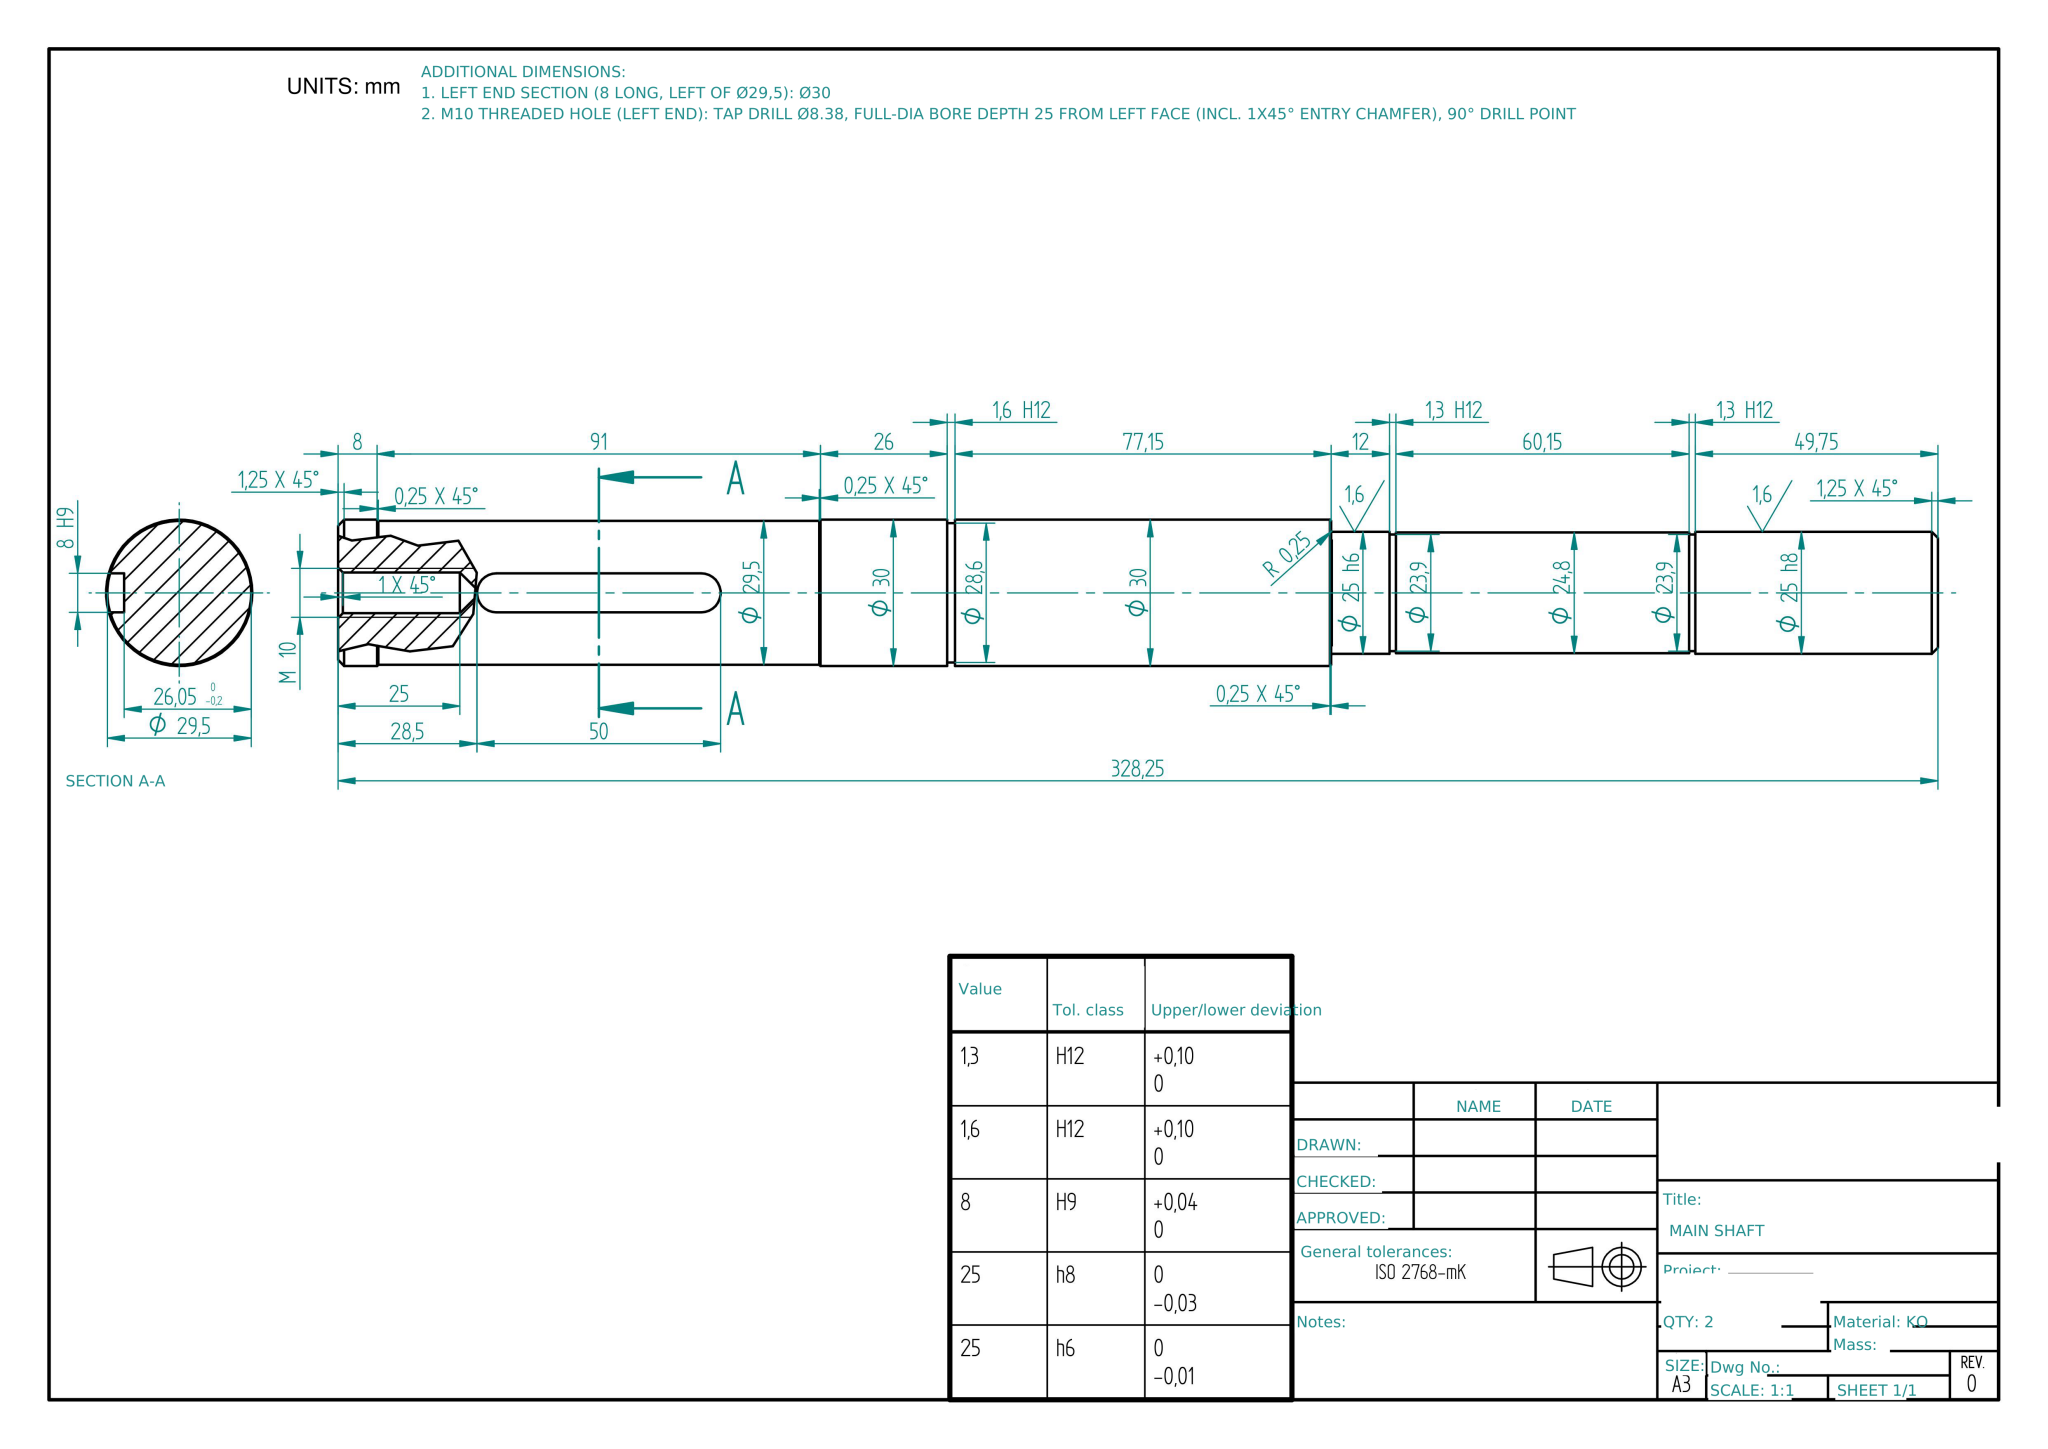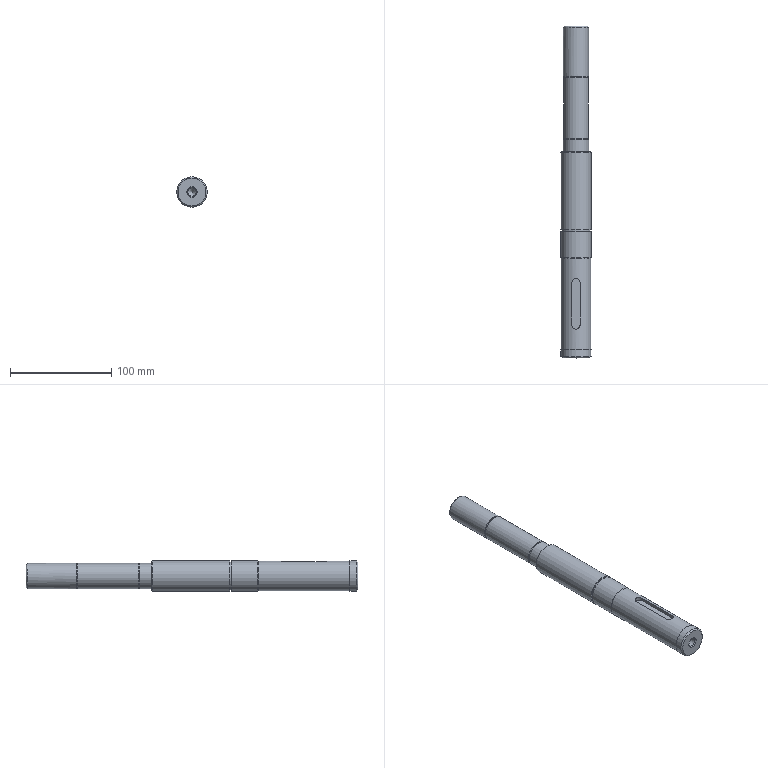Part | NX | mm | 1 solid | 33 faces | box 30 x 328.25 x 30 mm | volume 199467 mm3 | cylinder 13 | plane 12 | cone 7 | torus 1 | commonest cylinder face diameters 30 x3 8 x2 25 x2 23.9 x2 8.376 x1 29.5 x1 24.8 x1 28.6 x1
STEP:
#1=VALUE_REPRESENTATION_ITEM('',COUNT_MEASURE(0.));
#2=(LENGTH_UNIT()NAMED_UNIT(*)SI_UNIT(.MILLI.,.METRE.));
#3=UNCERTAINTY_MEASURE_WITH_UNIT(LENGTH_MEASURE(0.005),#2,'','');
#4=(NAMED_UNIT(*)PLANE_ANGLE_UNIT()SI_UNIT($,.RADIAN.));
#5=(NAMED_UNIT(*)SI_UNIT($,.STERADIAN.)SOLID_ANGLE_UNIT());
#6=(GEOMETRIC_REPRESENTATION_CONTEXT(3)GLOBAL_UNCERTAINTY_ASSIGNED_CONTEXT((#3))GLOBAL_UNIT_ASSIGNED_CONTEXT((#2,#4,#5))REPRESENTATION_CONTEXT('',''));
#7=REPRESENTATION('',(#1),#6);
#8=VALUE_REPRESENTATION_ITEM('',COUNT_MEASURE(0.));
#9=REPRESENTATION('',(#8),#6);
#10=CARTESIAN_POINT('',(0.,0.,0.));
#11=DIRECTION('',(0.,0.,1.));
#12=DIRECTION('',(1.,0.,0.));
#13=AXIS2_PLACEMENT_3D('',#10,#11,#12);
#14=SHAPE_REPRESENTATION('',(#13),#6);
#15=CARTESIAN_POINT('',(0.,-28.5,4.188));
#16=VERTEX_POINT('',#15);
#17=CARTESIAN_POINT('',(0.,-28.5,-0.));
#18=DIRECTION('',(0.,1.,0.));
#19=DIRECTION('',(0.,0.,1.));
#20=AXIS2_PLACEMENT_3D('',#17,#18,#19);
#21=CIRCLE('',#20,4.188);
#22=EDGE_CURVE('',#16,#16,#21,.T.);
#23=ORIENTED_EDGE('',*,*,#22,.F.);
#24=EDGE_LOOP('',(#23));
#25=FACE_BOUND('',#24,.T.);
#26=CARTESIAN_POINT('',(0.,-24.312,-0.));
#27=VERTEX_POINT('',#26);
#28=VERTEX_LOOP('',#27);
#29=FACE_BOUND('',#28,.T.);
#30=CARTESIAN_POINT('',(0.,-28.5,-0.));
#31=DIRECTION('',(0.,-1.,0.));
#32=DIRECTION('',(0.,0.,1.));
#33=AXIS2_PLACEMENT_3D('',#30,#31,#32);
#34=CONICAL_SURFACE('',#33,4.188,0.7854);
#35=ADVANCED_FACE('',(#25,#29),#34,.F.);
#36=CARTESIAN_POINT('',(0.,-53.5,5.188));
#37=VERTEX_POINT('',#36);
#38=CARTESIAN_POINT('',(0.,-53.5,-0.));
#39=DIRECTION('',(0.,1.,0.));
#40=DIRECTION('',(0.,0.,1.));
#41=AXIS2_PLACEMENT_3D('',#38,#39,#40);
#42=CIRCLE('',#41,5.188);
#43=EDGE_CURVE('',#37,#37,#42,.T.);
#44=ORIENTED_EDGE('',*,*,#43,.F.);
#45=EDGE_LOOP('',(#44));
#46=FACE_BOUND('',#45,.T.);
#47=CARTESIAN_POINT('',(0.,-52.5,4.188));
#48=VERTEX_POINT('',#47);
#49=CARTESIAN_POINT('',(0.,-52.5,-0.));
#50=DIRECTION('',(0.,-1.,0.));
#51=DIRECTION('',(0.,0.,1.));
#52=AXIS2_PLACEMENT_3D('',#49,#50,#51);
#53=CIRCLE('',#52,4.188);
#54=EDGE_CURVE('',#48,#48,#53,.T.);
#55=ORIENTED_EDGE('',*,*,#54,.F.);
#56=EDGE_LOOP('',(#55));
#57=FACE_BOUND('',#56,.T.);
#58=CARTESIAN_POINT('',(0.,-53.5,-0.));
#59=DIRECTION('',(0.,-1.,0.));
#60=DIRECTION('',(0.,0.,-1.));
#61=AXIS2_PLACEMENT_3D('',#58,#59,#60);
#62=CONICAL_SURFACE('',#61,5.188,0.7854);
#63=ADVANCED_FACE('',(#46,#57),#62,.F.);
#64=ORIENTED_EDGE('',*,*,#54,.T.);
#65=EDGE_LOOP('',(#64));
#66=FACE_BOUND('',#65,.T.);
#67=ORIENTED_EDGE('',*,*,#22,.T.);
#68=EDGE_LOOP('',(#67));
#69=FACE_BOUND('',#68,.T.);
#70=CARTESIAN_POINT('',(0.,-53.5,-0.));
#71=DIRECTION('',(0.,-1.,0.));
#72=DIRECTION('',(0.,0.,-1.));
#73=AXIS2_PLACEMENT_3D('',#70,#71,#72);
#74=CYLINDRICAL_SURFACE('',#73,4.188);
#75=ADVANCED_FACE('',(#66,#69),#74,.F.);
#76=CARTESIAN_POINT('',(-0.,-45.25,-14.75));
#77=VERTEX_POINT('',#76);
#78=CARTESIAN_POINT('',(-0.,-45.25,0.));
#79=DIRECTION('',(-0.,-1.,-0.));
#80=DIRECTION('',(0.,0.,-1.));
#81=AXIS2_PLACEMENT_3D('',#78,#79,#80);
#82=CIRCLE('',#81,14.75);
#83=EDGE_CURVE('',#77,#77,#82,.T.);
#84=ORIENTED_EDGE('',*,*,#83,.F.);
#85=EDGE_LOOP('',(#84));
#86=FACE_BOUND('',#85,.T.);
#87=CARTESIAN_POINT('',(0.,45.25,-14.75));
#88=VERTEX_POINT('',#87);
#89=CARTESIAN_POINT('',(0.,45.25,0.));
#90=DIRECTION('',(-0.,-1.,-0.));
#91=DIRECTION('',(0.,0.,-1.));
#92=AXIS2_PLACEMENT_3D('',#89,#90,#91);
#93=CIRCLE('',#92,14.75);
#94=EDGE_CURVE('',#88,#88,#93,.T.);
#95=ORIENTED_EDGE('',*,*,#94,.T.);
#96=EDGE_LOOP('',(#95));
#97=FACE_BOUND('',#96,.T.);
#98=CARTESIAN_POINT('',(-4.,21.,14.197));
#99=VERTEX_POINT('',#98);
#100=CARTESIAN_POINT('',(-4.,-21.,14.197));
#101=VERTEX_POINT('',#100);
#102=CARTESIAN_POINT('',(-4.,-60.,14.197));
#103=DIRECTION('',(-0.,-1.,-0.));
#104=VECTOR('',#103,1000.);
#105=LINE('',#102,#104);
#106=EDGE_CURVE('',#99,#101,#105,.T.);
#107=ORIENTED_EDGE('',*,*,#106,.F.);
#108=CARTESIAN_POINT('',(4.,21.,14.197));
#109=VERTEX_POINT('',#108);
#110=CARTESIAN_POINT('',(-4.,21.,14.197));
#111=CARTESIAN_POINT('',(-4.,22.062,14.197));
#112=CARTESIAN_POINT('',(-3.133,24.126,14.479));
#113=CARTESIAN_POINT('',(-0.005917,25.437,14.885));
#114=CARTESIAN_POINT('',(3.134,24.128,14.479));
#115=CARTESIAN_POINT('',(4.,22.062,14.197));
#116=CARTESIAN_POINT('',(4.,21.,14.197));
#117=B_SPLINE_CURVE_WITH_KNOTS('',3,(#110,#111,#112,#113,#114,#115,#116),.UNSPECIFIED.,.F.,.F.,(4,1,1,1,4),(0.,0.00314,0.00628,0.009421,0.01256),.UNSPECIFIED.);
#118=EDGE_CURVE('',#99,#109,#117,.T.);
#119=ORIENTED_EDGE('',*,*,#118,.T.);
#120=CARTESIAN_POINT('',(4.,-21.,14.197));
#121=VERTEX_POINT('',#120);
#122=CARTESIAN_POINT('',(4.,-60.,14.197));
#123=DIRECTION('',(0.,1.,0.));
#124=VECTOR('',#123,1000.);
#125=LINE('',#122,#124);
#126=EDGE_CURVE('',#121,#109,#125,.T.);
#127=ORIENTED_EDGE('',*,*,#126,.F.);
#128=CARTESIAN_POINT('',(4.,-21.,14.197));
#129=CARTESIAN_POINT('',(4.,-22.062,14.197));
#130=CARTESIAN_POINT('',(3.133,-24.126,14.479));
#131=CARTESIAN_POINT('',(0.005917,-25.437,14.885));
#132=CARTESIAN_POINT('',(-3.134,-24.128,14.479));
#133=CARTESIAN_POINT('',(-4.,-22.062,14.197));
#134=CARTESIAN_POINT('',(-4.,-21.,14.197));
#135=B_SPLINE_CURVE_WITH_KNOTS('',3,(#128,#129,#130,#131,#132,#133,#134),.UNSPECIFIED.,.F.,.F.,(4,1,1,1,4),(0.,0.00314,0.00628,0.009421,0.01256),.UNSPECIFIED.);
#136=EDGE_CURVE('',#121,#101,#135,.T.);
#137=ORIENTED_EDGE('',*,*,#136,.T.);
#138=EDGE_LOOP('',(#107,#119,#127,#137));
#139=FACE_BOUND('',#138,.T.);
#140=CARTESIAN_POINT('',(-0.,-60.,0.));
#141=DIRECTION('',(0.,1.,0.));
#142=DIRECTION('',(0.,0.,-1.));
#143=AXIS2_PLACEMENT_3D('',#140,#141,#142);
#144=CYLINDRICAL_SURFACE('',#143,14.75);
#145=ADVANCED_FACE('',(#86,#97,#139),#144,.T.);
#146=ORIENTED_EDGE('',*,*,#136,.F.);
#147=CARTESIAN_POINT('',(4.,-21.,11.3));
#148=VERTEX_POINT('',#147);
#149=CARTESIAN_POINT('',(4.,-21.,14.197));
#150=DIRECTION('',(0.,0.,1.));
#151=VECTOR('',#150,1000.);
#152=LINE('',#149,#151);
#153=EDGE_CURVE('',#148,#121,#152,.T.);
#154=ORIENTED_EDGE('',*,*,#153,.F.);
#155=CARTESIAN_POINT('',(-4.,-21.,11.3));
#156=VERTEX_POINT('',#155);
#157=CARTESIAN_POINT('',(0.,-21.,11.3));
#158=DIRECTION('',(0.,0.,1.));
#159=DIRECTION('',(1.,0.,0.));
#160=AXIS2_PLACEMENT_3D('',#157,#158,#159);
#161=CIRCLE('',#160,4.);
#162=EDGE_CURVE('',#156,#148,#161,.T.);
#163=ORIENTED_EDGE('',*,*,#162,.F.);
#164=CARTESIAN_POINT('',(-4.,-21.,11.3));
#165=DIRECTION('',(0.,0.,-1.));
#166=VECTOR('',#165,1000.);
#167=LINE('',#164,#166);
#168=EDGE_CURVE('',#101,#156,#167,.T.);
#169=ORIENTED_EDGE('',*,*,#168,.F.);
#170=EDGE_LOOP('',(#146,#154,#163,#169));
#171=FACE_BOUND('',#170,.T.);
#172=CARTESIAN_POINT('',(0.,-21.,270.792));
#173=DIRECTION('',(0.,0.,-1.));
#174=DIRECTION('',(1.,0.,0.));
#175=AXIS2_PLACEMENT_3D('',#172,#173,#174);
#176=CYLINDRICAL_SURFACE('',#175,4.);
#177=ADVANCED_FACE('',(#171),#176,.F.);
#178=CARTESIAN_POINT('',(0.,273.5,-12.5));
#179=VERTEX_POINT('',#178);
#180=CARTESIAN_POINT('',(0.,273.5,0.));
#181=DIRECTION('',(0.,-1.,0.));
#182=DIRECTION('',(0.,0.,-1.));
#183=AXIS2_PLACEMENT_3D('',#180,#181,#182);
#184=CIRCLE('',#183,12.5);
#185=EDGE_CURVE('',#179,#179,#184,.T.);
#186=ORIENTED_EDGE('',*,*,#185,.F.);
#187=EDGE_LOOP('',(#186));
#188=FACE_BOUND('',#187,.T.);
#189=CARTESIAN_POINT('',(0.,274.75,-11.25));
#190=VERTEX_POINT('',#189);
#191=CARTESIAN_POINT('',(0.,274.75,0.));
#192=DIRECTION('',(0.,1.,0.));
#193=DIRECTION('',(0.,0.,-1.));
#194=AXIS2_PLACEMENT_3D('',#191,#192,#193);
#195=CIRCLE('',#194,11.25);
#196=EDGE_CURVE('',#190,#190,#195,.T.);
#197=ORIENTED_EDGE('',*,*,#196,.F.);
#198=EDGE_LOOP('',(#197));
#199=FACE_BOUND('',#198,.T.);
#200=CARTESIAN_POINT('',(0.,273.5,0.));
#201=DIRECTION('',(0.,-1.,0.));
#202=DIRECTION('',(0.,0.,-1.));
#203=AXIS2_PLACEMENT_3D('',#200,#201,#202);
#204=CONICAL_SURFACE('',#203,12.5,0.7854);
#205=ADVANCED_FACE('',(#188,#199),#204,.T.);
#206=CARTESIAN_POINT('',(12.5,225.,0.));
#207=VERTEX_POINT('',#206);
#208=CARTESIAN_POINT('',(0.,225.,0.));
#209=DIRECTION('',(-0.,-1.,0.));
#210=DIRECTION('',(1.,-0.,0.));
#211=AXIS2_PLACEMENT_3D('',#208,#209,#210);
#212=CIRCLE('',#211,12.5);
#213=EDGE_CURVE('',#207,#207,#212,.T.);
#214=ORIENTED_EDGE('',*,*,#213,.F.);
#215=EDGE_LOOP('',(#214));
#216=FACE_BOUND('',#215,.T.);
#217=ORIENTED_EDGE('',*,*,#185,.T.);
#218=EDGE_LOOP('',(#217));
#219=FACE_BOUND('',#218,.T.);
#220=CARTESIAN_POINT('',(0.,150.25,0.));
#221=DIRECTION('',(0.,-1.,0.));
#222=DIRECTION('',(0.,0.,1.));
#223=AXIS2_PLACEMENT_3D('',#220,#221,#222);
#224=CYLINDRICAL_SURFACE('',#223,12.5);
#225=ADVANCED_FACE('',(#216,#219),#224,.T.);
#226=ORIENTED_EDGE('',*,*,#196,.T.);
#227=EDGE_LOOP('',(#226));
#228=FACE_BOUND('',#227,.T.);
#229=CARTESIAN_POINT('',(0.,274.75,0.));
#230=DIRECTION('',(0.,-1.,0.));
#231=DIRECTION('',(0.,0.,-1.));
#232=AXIS2_PLACEMENT_3D('',#229,#230,#231);
#233=PLANE('',#232);
#234=ADVANCED_FACE('',(#228),#233,.F.);
#235=CARTESIAN_POINT('',(0.,-52.25,15.));
#236=VERTEX_POINT('',#235);
#237=CARTESIAN_POINT('',(0.,-52.25,0.));
#238=DIRECTION('',(0.,1.,0.));
#239=DIRECTION('',(0.,0.,1.));
#240=AXIS2_PLACEMENT_3D('',#237,#238,#239);
#241=CIRCLE('',#240,15.);
#242=EDGE_CURVE('',#236,#236,#241,.T.);
#243=ORIENTED_EDGE('',*,*,#242,.F.);
#244=EDGE_LOOP('',(#243));
#245=FACE_BOUND('',#244,.T.);
#246=CARTESIAN_POINT('',(0.,-53.5,13.75));
#247=VERTEX_POINT('',#246);
#248=CARTESIAN_POINT('',(0.,-53.5,0.));
#249=DIRECTION('',(0.,-1.,0.));
#250=DIRECTION('',(0.,0.,1.));
#251=AXIS2_PLACEMENT_3D('',#248,#249,#250);
#252=CIRCLE('',#251,13.75);
#253=EDGE_CURVE('',#247,#247,#252,.T.);
#254=ORIENTED_EDGE('',*,*,#253,.F.);
#255=EDGE_LOOP('',(#254));
#256=FACE_BOUND('',#255,.T.);
#257=CARTESIAN_POINT('',(0.,-52.25,0.));
#258=DIRECTION('',(0.,1.,0.));
#259=DIRECTION('',(0.,0.,1.));
#260=AXIS2_PLACEMENT_3D('',#257,#258,#259);
#261=CONICAL_SURFACE('',#260,15.,0.7854);
#262=ADVANCED_FACE('',(#245,#256),#261,.T.);
#263=CARTESIAN_POINT('',(0.,-45.5,-15.));
#264=VERTEX_POINT('',#263);
#265=CARTESIAN_POINT('',(0.,-45.5,0.));
#266=DIRECTION('',(0.,-1.,0.));
#267=DIRECTION('',(0.,0.,-1.));
#268=AXIS2_PLACEMENT_3D('',#265,#266,#267);
#269=CIRCLE('',#268,15.);
#270=EDGE_CURVE('',#264,#264,#269,.T.);
#271=ORIENTED_EDGE('',*,*,#270,.T.);
#272=EDGE_LOOP('',(#271));
#273=FACE_BOUND('',#272,.T.);
#274=ORIENTED_EDGE('',*,*,#242,.T.);
#275=EDGE_LOOP('',(#274));
#276=FACE_BOUND('',#275,.T.);
#277=CARTESIAN_POINT('',(0.,202.5,0.));
#278=DIRECTION('',(0.,1.,0.));
#279=DIRECTION('',(0.,0.,-1.));
#280=AXIS2_PLACEMENT_3D('',#277,#278,#279);
#281=CYLINDRICAL_SURFACE('',#280,15.);
#282=ADVANCED_FACE('',(#273,#276),#281,.T.);
#283=ORIENTED_EDGE('',*,*,#106,.T.);
#284=ORIENTED_EDGE('',*,*,#168,.T.);
#285=CARTESIAN_POINT('',(-4.,21.,11.3));
#286=VERTEX_POINT('',#285);
#287=CARTESIAN_POINT('',(-4.,25.,11.3));
#288=DIRECTION('',(0.,-1.,0.));
#289=VECTOR('',#288,1000.);
#290=LINE('',#287,#289);
#291=EDGE_CURVE('',#286,#156,#290,.T.);
#292=ORIENTED_EDGE('',*,*,#291,.F.);
#293=CARTESIAN_POINT('',(-4.,21.,14.197));
#294=DIRECTION('',(0.,0.,1.));
#295=VECTOR('',#294,1000.);
#296=LINE('',#293,#295);
#297=EDGE_CURVE('',#286,#99,#296,.T.);
#298=ORIENTED_EDGE('',*,*,#297,.T.);
#299=EDGE_LOOP('',(#283,#284,#292,#298));
#300=FACE_BOUND('',#299,.T.);
#301=CARTESIAN_POINT('',(-4.,25.,270.792));
#302=DIRECTION('',(1.,0.,0.));
#303=DIRECTION('',(0.,1.,0.));
#304=AXIS2_PLACEMENT_3D('',#301,#302,#303);
#305=PLANE('',#304);
#306=ADVANCED_FACE('',(#300),#305,.T.);
#307=ORIENTED_EDGE('',*,*,#126,.T.);
#308=CARTESIAN_POINT('',(4.,21.,11.3));
#309=VERTEX_POINT('',#308);
#310=CARTESIAN_POINT('',(4.,21.,11.3));
#311=DIRECTION('',(0.,0.,-1.));
#312=VECTOR('',#311,1000.);
#313=LINE('',#310,#312);
#314=EDGE_CURVE('',#109,#309,#313,.T.);
#315=ORIENTED_EDGE('',*,*,#314,.T.);
#316=CARTESIAN_POINT('',(4.,-25.,11.3));
#317=DIRECTION('',(0.,1.,0.));
#318=VECTOR('',#317,1000.);
#319=LINE('',#316,#318);
#320=EDGE_CURVE('',#148,#309,#319,.T.);
#321=ORIENTED_EDGE('',*,*,#320,.F.);
#322=ORIENTED_EDGE('',*,*,#153,.T.);
#323=EDGE_LOOP('',(#307,#315,#321,#322));
#324=FACE_BOUND('',#323,.T.);
#325=CARTESIAN_POINT('',(4.,-25.,270.792));
#326=DIRECTION('',(-1.,0.,0.));
#327=DIRECTION('',(0.,0.,1.));
#328=AXIS2_PLACEMENT_3D('',#325,#326,#327);
#329=PLANE('',#328);
#330=ADVANCED_FACE('',(#324),#329,.T.);
#331=CARTESIAN_POINT('',(0.,150.,15.));
#332=VERTEX_POINT('',#331);
#333=CARTESIAN_POINT('',(0.,150.,0.));
#334=DIRECTION('',(0.,-1.,0.));
#335=DIRECTION('',(0.,0.,1.));
#336=AXIS2_PLACEMENT_3D('',#333,#334,#335);
#337=CIRCLE('',#336,15.);
#338=EDGE_CURVE('',#332,#332,#337,.T.);
#339=ORIENTED_EDGE('',*,*,#338,.F.);
#340=EDGE_LOOP('',(#339));
#341=FACE_BOUND('',#340,.T.);
#342=CARTESIAN_POINT('',(0.,150.25,14.75));
#343=VERTEX_POINT('',#342);
#344=CARTESIAN_POINT('',(0.,150.25,0.));
#345=DIRECTION('',(0.,1.,0.));
#346=DIRECTION('',(0.,0.,1.));
#347=AXIS2_PLACEMENT_3D('',#344,#345,#346);
#348=CIRCLE('',#347,14.75);
#349=EDGE_CURVE('',#343,#343,#348,.T.);
#350=ORIENTED_EDGE('',*,*,#349,.F.);
#351=EDGE_LOOP('',(#350));
#352=FACE_BOUND('',#351,.T.);
#353=CARTESIAN_POINT('',(0.,150.25,0.));
#354=DIRECTION('',(0.,-1.,0.));
#355=DIRECTION('',(0.,0.,-1.));
#356=AXIS2_PLACEMENT_3D('',#353,#354,#355);
#357=CONICAL_SURFACE('',#356,14.75,0.7854);
#358=ADVANCED_FACE('',(#341,#352),#357,.T.);
#359=ORIENTED_EDGE('',*,*,#320,.T.);
#360=CARTESIAN_POINT('',(0.,21.,11.3));
#361=DIRECTION('',(0.,0.,1.));
#362=DIRECTION('',(1.,0.,0.));
#363=AXIS2_PLACEMENT_3D('',#360,#361,#362);
#364=CIRCLE('',#363,4.);
#365=EDGE_CURVE('',#309,#286,#364,.T.);
#366=ORIENTED_EDGE('',*,*,#365,.T.);
#367=ORIENTED_EDGE('',*,*,#291,.T.);
#368=ORIENTED_EDGE('',*,*,#162,.T.);
#369=EDGE_LOOP('',(#359,#366,#367,#368));
#370=FACE_BOUND('',#369,.T.);
#371=CARTESIAN_POINT('',(-4.,-25.,11.3));
#372=DIRECTION('',(0.,0.,1.));
#373=DIRECTION('',(1.,0.,0.));
#374=AXIS2_PLACEMENT_3D('',#371,#372,#373);
#375=PLANE('',#374);
#376=ADVANCED_FACE('',(#370),#375,.T.);
#377=CARTESIAN_POINT('',(0.,223.7,-12.4));
#378=VERTEX_POINT('',#377);
#379=CARTESIAN_POINT('',(0.,223.7,0.));
#380=DIRECTION('',(-0.,-1.,-0.));
#381=DIRECTION('',(0.,0.,-1.));
#382=AXIS2_PLACEMENT_3D('',#379,#380,#381);
#383=CIRCLE('',#382,12.4);
#384=EDGE_CURVE('',#378,#378,#383,.T.);
#385=ORIENTED_EDGE('',*,*,#384,.F.);
#386=EDGE_LOOP('',(#385));
#387=FACE_BOUND('',#386,.T.);
#388=CARTESIAN_POINT('',(11.95,223.7,0.));
#389=VERTEX_POINT('',#388);
#390=CARTESIAN_POINT('',(0.,223.7,0.));
#391=DIRECTION('',(-0.,-1.,0.));
#392=DIRECTION('',(1.,-0.,0.));
#393=AXIS2_PLACEMENT_3D('',#390,#391,#392);
#394=CIRCLE('',#393,11.95);
#395=EDGE_CURVE('',#389,#389,#394,.T.);
#396=ORIENTED_EDGE('',*,*,#395,.T.);
#397=EDGE_LOOP('',(#396));
#398=FACE_BOUND('',#397,.T.);
#399=CARTESIAN_POINT('',(-21.95,223.7,0.));
#400=DIRECTION('',(0.,1.,0.));
#401=DIRECTION('',(1.,0.,-0.));
#402=AXIS2_PLACEMENT_3D('',#399,#400,#401);
#403=PLANE('',#402);
#404=ADVANCED_FACE('',(#387,#398),#403,.T.);
#405=ORIENTED_EDGE('',*,*,#395,.F.);
#406=EDGE_LOOP('',(#405));
#407=FACE_BOUND('',#406,.T.);
#408=CARTESIAN_POINT('',(11.95,225.,0.));
#409=VERTEX_POINT('',#408);
#410=CARTESIAN_POINT('',(0.,225.,0.));
#411=DIRECTION('',(-0.,-1.,0.));
#412=DIRECTION('',(1.,-0.,0.));
#413=AXIS2_PLACEMENT_3D('',#410,#411,#412);
#414=CIRCLE('',#413,11.95);
#415=EDGE_CURVE('',#409,#409,#414,.T.);
#416=ORIENTED_EDGE('',*,*,#415,.T.);
#417=EDGE_LOOP('',(#416));
#418=FACE_BOUND('',#417,.T.);
#419=CARTESIAN_POINT('',(0.,54.,0.));
#420=DIRECTION('',(0.,1.,0.));
#421=DIRECTION('',(1.,-0.,0.));
#422=AXIS2_PLACEMENT_3D('',#419,#420,#421);
#423=CYLINDRICAL_SURFACE('',#422,11.95);
#424=ADVANCED_FACE('',(#407,#418),#423,.T.);
#425=ORIENTED_EDGE('',*,*,#213,.T.);
#426=EDGE_LOOP('',(#425));
#427=FACE_BOUND('',#426,.T.);
#428=ORIENTED_EDGE('',*,*,#415,.F.);
#429=EDGE_LOOP('',(#428));
#430=FACE_BOUND('',#429,.T.);
#431=CARTESIAN_POINT('',(-21.95,225.,0.));
#432=DIRECTION('',(-0.,-1.,0.));
#433=DIRECTION('',(-1.,0.,0.));
#434=AXIS2_PLACEMENT_3D('',#431,#432,#433);
#435=PLANE('',#434);
#436=ADVANCED_FACE('',(#427,#430),#435,.T.);
#437=ORIENTED_EDGE('',*,*,#384,.T.);
#438=EDGE_LOOP('',(#437));
#439=FACE_BOUND('',#438,.T.);
#440=CARTESIAN_POINT('',(0.,163.55,-12.4));
#441=VERTEX_POINT('',#440);
#442=CARTESIAN_POINT('',(0.,163.55,0.));
#443=DIRECTION('',(-0.,-1.,-0.));
#444=DIRECTION('',(0.,0.,-1.));
#445=AXIS2_PLACEMENT_3D('',#442,#443,#444);
#446=CIRCLE('',#445,12.4);
#447=EDGE_CURVE('',#441,#441,#446,.T.);
#448=ORIENTED_EDGE('',*,*,#447,.F.);
#449=EDGE_LOOP('',(#448));
#450=FACE_BOUND('',#449,.T.);
#451=CARTESIAN_POINT('',(-0.,-60.,0.));
#452=DIRECTION('',(0.,1.,0.));
#453=DIRECTION('',(0.,0.,-1.));
#454=AXIS2_PLACEMENT_3D('',#451,#452,#453);
#455=CYLINDRICAL_SURFACE('',#454,12.4);
#456=ADVANCED_FACE('',(#439,#450),#455,.T.);
#457=CARTESIAN_POINT('',(0.,73.1,-15.));
#458=VERTEX_POINT('',#457);
#459=CARTESIAN_POINT('',(0.,73.1,0.));
#460=DIRECTION('',(-0.,-1.,-0.));
#461=DIRECTION('',(0.,0.,-1.));
#462=AXIS2_PLACEMENT_3D('',#459,#460,#461);
#463=CIRCLE('',#462,15.);
#464=EDGE_CURVE('',#458,#458,#463,.T.);
#465=ORIENTED_EDGE('',*,*,#464,.T.);
#466=EDGE_LOOP('',(#465));
#467=FACE_BOUND('',#466,.T.);
#468=CARTESIAN_POINT('',(0.,73.1,-14.3));
#469=VERTEX_POINT('',#468);
#470=CARTESIAN_POINT('',(0.,73.1,0.));
#471=DIRECTION('',(-0.,-1.,-0.));
#472=DIRECTION('',(0.,0.,-1.));
#473=AXIS2_PLACEMENT_3D('',#470,#471,#472);
#474=CIRCLE('',#473,14.3);
#475=EDGE_CURVE('',#469,#469,#474,.T.);
#476=ORIENTED_EDGE('',*,*,#475,.F.);
#477=EDGE_LOOP('',(#476));
#478=FACE_BOUND('',#477,.T.);
#479=CARTESIAN_POINT('',(0.,73.1,14.3));
#480=DIRECTION('',(-0.,-1.,-0.));
#481=DIRECTION('',(0.,0.,-1.));
#482=AXIS2_PLACEMENT_3D('',#479,#480,#481);
#483=PLANE('',#482);
#484=ADVANCED_FACE('',(#467,#478),#483,.T.);
#485=CARTESIAN_POINT('',(0.,71.5,-15.));
#486=VERTEX_POINT('',#485);
#487=CARTESIAN_POINT('',(0.,71.5,0.));
#488=DIRECTION('',(-0.,-1.,-0.));
#489=DIRECTION('',(0.,0.,-1.));
#490=AXIS2_PLACEMENT_3D('',#487,#488,#489);
#491=CIRCLE('',#490,15.);
#492=EDGE_CURVE('',#486,#486,#491,.T.);
#493=ORIENTED_EDGE('',*,*,#492,.T.);
#494=EDGE_LOOP('',(#493));
#495=FACE_BOUND('',#494,.T.);
#496=CARTESIAN_POINT('',(0.,45.5,15.));
#497=VERTEX_POINT('',#496);
#498=CARTESIAN_POINT('',(0.,45.5,0.));
#499=DIRECTION('',(0.,1.,0.));
#500=DIRECTION('',(0.,0.,1.));
#501=AXIS2_PLACEMENT_3D('',#498,#499,#500);
#502=CIRCLE('',#501,15.);
#503=EDGE_CURVE('',#497,#497,#502,.T.);
#504=ORIENTED_EDGE('',*,*,#503,.T.);
#505=EDGE_LOOP('',(#504));
#506=FACE_BOUND('',#505,.T.);
#507=CARTESIAN_POINT('',(0.,202.5,0.));
#508=DIRECTION('',(0.,1.,0.));
#509=DIRECTION('',(0.,0.,-1.));
#510=AXIS2_PLACEMENT_3D('',#507,#508,#509);
#511=CYLINDRICAL_SURFACE('',#510,15.);
#512=ADVANCED_FACE('',(#495,#506),#511,.T.);
#513=CARTESIAN_POINT('',(0.,71.5,-14.3));
#514=VERTEX_POINT('',#513);
#515=CARTESIAN_POINT('',(0.,71.5,0.));
#516=DIRECTION('',(-0.,-1.,-0.));
#517=DIRECTION('',(0.,0.,-1.));
#518=AXIS2_PLACEMENT_3D('',#515,#516,#517);
#519=CIRCLE('',#518,14.3);
#520=EDGE_CURVE('',#514,#514,#519,.T.);
#521=ORIENTED_EDGE('',*,*,#520,.F.);
#522=EDGE_LOOP('',(#521));
#523=FACE_BOUND('',#522,.T.);
#524=ORIENTED_EDGE('',*,*,#475,.T.);
#525=EDGE_LOOP('',(#524));
#526=FACE_BOUND('',#525,.T.);
#527=CARTESIAN_POINT('',(-0.,-60.,0.));
#528=DIRECTION('',(0.,1.,0.));
#529=DIRECTION('',(0.,0.,-1.));
#530=AXIS2_PLACEMENT_3D('',#527,#528,#529);
#531=CYLINDRICAL_SURFACE('',#530,14.3);
#532=ADVANCED_FACE('',(#523,#526),#531,.T.);
#533=ORIENTED_EDGE('',*,*,#492,.F.);
#534=EDGE_LOOP('',(#533));
#535=FACE_BOUND('',#534,.T.);
#536=ORIENTED_EDGE('',*,*,#520,.T.);
#537=EDGE_LOOP('',(#536));
#538=FACE_BOUND('',#537,.T.);
#539=CARTESIAN_POINT('',(0.,71.5,15.));
#540=DIRECTION('',(0.,1.,0.));
#541=DIRECTION('',(1.,0.,-0.));
#542=AXIS2_PLACEMENT_3D('',#539,#540,#541);
#543=PLANE('',#542);
#544=ADVANCED_FACE('',(#535,#538),#543,.T.);
#545=ORIENTED_EDGE('',*,*,#349,.T.);
#546=EDGE_LOOP('',(#545));
#547=FACE_BOUND('',#546,.T.);
#548=CARTESIAN_POINT('',(0.,150.25,12.75));
#549=VERTEX_POINT('',#548);
#550=CARTESIAN_POINT('',(0.,150.25,0.));
#551=DIRECTION('',(0.,-1.,0.));
#552=DIRECTION('',(0.,0.,1.));
#553=AXIS2_PLACEMENT_3D('',#550,#551,#552);
#554=CIRCLE('',#553,12.75);
#555=EDGE_CURVE('',#549,#549,#554,.T.);
#556=ORIENTED_EDGE('',*,*,#555,.T.);
#557=EDGE_LOOP('',(#556));
#558=FACE_BOUND('',#557,.T.);
#559=CARTESIAN_POINT('',(-6.25,150.25,0.));
#560=DIRECTION('',(0.,1.,0.));
#561=DIRECTION('',(1.,0.,0.));
#562=AXIS2_PLACEMENT_3D('',#559,#560,#561);
#563=PLANE('',#562);
#564=ADVANCED_FACE('',(#547,#558),#563,.T.);
#565=ORIENTED_EDGE('',*,*,#253,.T.);
#566=EDGE_LOOP('',(#565));
#567=FACE_BOUND('',#566,.T.);
#568=ORIENTED_EDGE('',*,*,#43,.T.);
#569=EDGE_LOOP('',(#568));
#570=FACE_BOUND('',#569,.T.);
#571=CARTESIAN_POINT('',(0.,-53.5,0.));
#572=DIRECTION('',(0.,1.,0.));
#573=DIRECTION('',(1.,0.,0.));
#574=AXIS2_PLACEMENT_3D('',#571,#572,#573);
#575=PLANE('',#574);
#576=ADVANCED_FACE('',(#567,#570),#575,.F.);
#577=ORIENTED_EDGE('',*,*,#270,.F.);
#578=EDGE_LOOP('',(#577));
#579=FACE_BOUND('',#578,.T.);
#580=ORIENTED_EDGE('',*,*,#83,.T.);
#581=EDGE_LOOP('',(#580));
#582=FACE_BOUND('',#581,.T.);
#583=CARTESIAN_POINT('',(0.,-45.5,0.));
#584=DIRECTION('',(0.,-1.,0.));
#585=DIRECTION('',(0.,0.,-1.));
#586=AXIS2_PLACEMENT_3D('',#583,#584,#585);
#587=CONICAL_SURFACE('',#586,15.,0.7854);
#588=ADVANCED_FACE('',(#579,#582),#587,.T.);
#589=ORIENTED_EDGE('',*,*,#503,.F.);
#590=EDGE_LOOP('',(#589));
#591=FACE_BOUND('',#590,.T.);
#592=ORIENTED_EDGE('',*,*,#94,.F.);
#593=EDGE_LOOP('',(#592));
#594=FACE_BOUND('',#593,.T.);
#595=CARTESIAN_POINT('',(0.,45.25,0.));
#596=DIRECTION('',(0.,1.,0.));
#597=DIRECTION('',(0.,0.,1.));
#598=AXIS2_PLACEMENT_3D('',#595,#596,#597);
#599=CONICAL_SURFACE('',#598,14.75,0.7854);
#600=ADVANCED_FACE('',(#591,#594),#599,.T.);
#601=ORIENTED_EDGE('',*,*,#555,.F.);
#602=EDGE_LOOP('',(#601));
#603=FACE_BOUND('',#602,.T.);
#604=CARTESIAN_POINT('',(0.,150.5,12.5));
#605=VERTEX_POINT('',#604);
#606=CARTESIAN_POINT('',(0.,150.5,0.));
#607=DIRECTION('',(0.,1.,0.));
#608=DIRECTION('',(0.,0.,1.));
#609=AXIS2_PLACEMENT_3D('',#606,#607,#608);
#610=CIRCLE('',#609,12.5);
#611=EDGE_CURVE('',#605,#605,#610,.T.);
#612=ORIENTED_EDGE('',*,*,#611,.F.);
#613=EDGE_LOOP('',(#612));
#614=FACE_BOUND('',#613,.T.);
#615=CARTESIAN_POINT('',(0.,150.5,0.));
#616=DIRECTION('',(0.,1.,0.));
#617=DIRECTION('',(0.,0.,1.));
#618=AXIS2_PLACEMENT_3D('',#615,#616,#617);
#619=TOROIDAL_SURFACE('',#618,12.75,0.25);
#620=ADVANCED_FACE('',(#603,#614),#619,.F.);
#621=CARTESIAN_POINT('',(0.,162.25,-12.5));
#622=VERTEX_POINT('',#621);
#623=CARTESIAN_POINT('',(0.,162.25,0.));
#624=DIRECTION('',(-0.,-1.,-0.));
#625=DIRECTION('',(0.,0.,-1.));
#626=AXIS2_PLACEMENT_3D('',#623,#624,#625);
#627=CIRCLE('',#626,12.5);
#628=EDGE_CURVE('',#622,#622,#627,.T.);
#629=ORIENTED_EDGE('',*,*,#628,.T.);
#630=EDGE_LOOP('',(#629));
#631=FACE_BOUND('',#630,.T.);
#632=ORIENTED_EDGE('',*,*,#611,.T.);
#633=EDGE_LOOP('',(#632));
#634=FACE_BOUND('',#633,.T.);
#635=CARTESIAN_POINT('',(0.,150.25,0.));
#636=DIRECTION('',(0.,-1.,0.));
#637=DIRECTION('',(0.,0.,1.));
#638=AXIS2_PLACEMENT_3D('',#635,#636,#637);
#639=CYLINDRICAL_SURFACE('',#638,12.5);
#640=ADVANCED_FACE('',(#631,#634),#639,.T.);
#641=ORIENTED_EDGE('',*,*,#628,.F.);
#642=EDGE_LOOP('',(#641));
#643=FACE_BOUND('',#642,.T.);
#644=CARTESIAN_POINT('',(0.,162.25,-11.95));
#645=VERTEX_POINT('',#644);
#646=CARTESIAN_POINT('',(0.,162.25,0.));
#647=DIRECTION('',(-0.,-1.,-0.));
#648=DIRECTION('',(0.,0.,-1.));
#649=AXIS2_PLACEMENT_3D('',#646,#647,#648);
#650=CIRCLE('',#649,11.95);
#651=EDGE_CURVE('',#645,#645,#650,.T.);
#652=ORIENTED_EDGE('',*,*,#651,.T.);
#653=EDGE_LOOP('',(#652));
#654=FACE_BOUND('',#653,.T.);
#655=CARTESIAN_POINT('',(0.,162.25,11.95));
#656=DIRECTION('',(-0.,-1.,-0.));
#657=DIRECTION('',(0.,0.,-1.));
#658=AXIS2_PLACEMENT_3D('',#655,#656,#657);
#659=PLANE('',#658);
#660=ADVANCED_FACE('',(#643,#654),#659,.F.);
#661=CARTESIAN_POINT('',(0.,163.55,-11.95));
#662=VERTEX_POINT('',#661);
#663=CARTESIAN_POINT('',(0.,163.55,0.));
#664=DIRECTION('',(-0.,-1.,-0.));
#665=DIRECTION('',(0.,0.,-1.));
#666=AXIS2_PLACEMENT_3D('',#663,#664,#665);
#667=CIRCLE('',#666,11.95);
#668=EDGE_CURVE('',#662,#662,#667,.T.);
#669=ORIENTED_EDGE('',*,*,#668,.T.);
#670=EDGE_LOOP('',(#669));
#671=FACE_BOUND('',#670,.T.);
#672=ORIENTED_EDGE('',*,*,#651,.F.);
#673=EDGE_LOOP('',(#672));
#674=FACE_BOUND('',#673,.T.);
#675=CARTESIAN_POINT('',(-0.,-60.,0.));
#676=DIRECTION('',(0.,1.,0.));
#677=DIRECTION('',(0.,0.,-1.));
#678=AXIS2_PLACEMENT_3D('',#675,#676,#677);
#679=CYLINDRICAL_SURFACE('',#678,11.95);
#680=ADVANCED_FACE('',(#671,#674),#679,.T.);
#681=ORIENTED_EDGE('',*,*,#447,.T.);
#682=EDGE_LOOP('',(#681));
#683=FACE_BOUND('',#682,.T.);
#684=ORIENTED_EDGE('',*,*,#668,.F.);
#685=EDGE_LOOP('',(#684));
#686=FACE_BOUND('',#685,.T.);
#687=CARTESIAN_POINT('',(0.,163.55,12.5));
#688=DIRECTION('',(0.,1.,0.));
#689=DIRECTION('',(1.,0.,-0.));
#690=AXIS2_PLACEMENT_3D('',#687,#688,#689);
#691=PLANE('',#690);
#692=ADVANCED_FACE('',(#683,#686),#691,.F.);
#693=ORIENTED_EDGE('',*,*,#118,.F.);
#694=ORIENTED_EDGE('',*,*,#297,.F.);
#695=ORIENTED_EDGE('',*,*,#365,.F.);
#696=ORIENTED_EDGE('',*,*,#314,.F.);
#697=EDGE_LOOP('',(#693,#694,#695,#696));
#698=FACE_BOUND('',#697,.T.);
#699=CARTESIAN_POINT('',(0.,21.,270.792));
#700=DIRECTION('',(0.,0.,-1.));
#701=DIRECTION('',(1.,0.,0.));
#702=AXIS2_PLACEMENT_3D('',#699,#700,#701);
#703=CYLINDRICAL_SURFACE('',#702,4.);
#704=ADVANCED_FACE('',(#698),#703,.F.);
#705=ORIENTED_EDGE('',*,*,#464,.F.);
#706=EDGE_LOOP('',(#705));
#707=FACE_BOUND('',#706,.T.);
#708=ORIENTED_EDGE('',*,*,#338,.T.);
#709=EDGE_LOOP('',(#708));
#710=FACE_BOUND('',#709,.T.);
#711=CARTESIAN_POINT('',(0.,202.5,0.));
#712=DIRECTION('',(0.,1.,0.));
#713=DIRECTION('',(0.,0.,-1.));
#714=AXIS2_PLACEMENT_3D('',#711,#712,#713);
#715=CYLINDRICAL_SURFACE('',#714,15.);
#716=ADVANCED_FACE('',(#707,#710),#715,.T.);
#717=CLOSED_SHELL('',(#35,#63,#75,#145,#177,#205,#225,#234,#262,#282,#306,#330,#358,#376,#404,#424,#436,#456,#484,#512,#532,#544,#564,#576,#588,#600,#620,#640,#660,#680,#692,#704,#716));
#718=MANIFOLD_SOLID_BREP('',#717);
#719=ADVANCED_BREP_SHAPE_REPRESENTATION('',(#718),#6);
#720=SHAPE_REPRESENTATION_RELATIONSHIP('','',#14,#719);
#721=COLOUR_RGB('',0.8,0.8,0.8);
#722=FILL_AREA_STYLE_COLOUR('',#721);
#723=FILL_AREA_STYLE('',(#722));
#724=SURFACE_STYLE_FILL_AREA(#723);
#725=SURFACE_SIDE_STYLE('',(#724));
#726=SURFACE_STYLE_USAGE(.BOTH.,#725);
#727=PRESENTATION_STYLE_ASSIGNMENT((#726));
#728=STYLED_ITEM('',(#727),#35);
#729=FILL_AREA_STYLE_COLOUR('',#721);
#730=FILL_AREA_STYLE('',(#729));
#731=SURFACE_STYLE_FILL_AREA(#730);
#732=SURFACE_SIDE_STYLE('',(#731));
#733=SURFACE_STYLE_USAGE(.BOTH.,#732);
#734=PRESENTATION_STYLE_ASSIGNMENT((#733));
#735=STYLED_ITEM('',(#734),#63);
#736=COLOUR_RGB('',0.6452,0.6789,0.7);
#737=FILL_AREA_STYLE_COLOUR('',#736);
#738=FILL_AREA_STYLE('',(#737));
#739=SURFACE_STYLE_FILL_AREA(#738);
#740=SURFACE_SIDE_STYLE('',(#739));
#741=SURFACE_STYLE_USAGE(.BOTH.,#740);
#742=PRESENTATION_STYLE_ASSIGNMENT((#741));
#743=STYLED_ITEM('',(#742),#75);
#744=FILL_AREA_STYLE_COLOUR('',#721);
#745=FILL_AREA_STYLE('',(#744));
#746=SURFACE_STYLE_FILL_AREA(#745);
#747=SURFACE_SIDE_STYLE('',(#746));
#748=SURFACE_STYLE_USAGE(.BOTH.,#747);
#749=PRESENTATION_STYLE_ASSIGNMENT((#748));
#750=STYLED_ITEM('',(#749),#145);
#751=FILL_AREA_STYLE_COLOUR('',#721);
#752=FILL_AREA_STYLE('',(#751));
#753=SURFACE_STYLE_FILL_AREA(#752);
#754=SURFACE_SIDE_STYLE('',(#753));
#755=SURFACE_STYLE_USAGE(.BOTH.,#754);
#756=PRESENTATION_STYLE_ASSIGNMENT((#755));
#757=STYLED_ITEM('',(#756),#177);
#758=FILL_AREA_STYLE_COLOUR('',#721);
#759=FILL_AREA_STYLE('',(#758));
#760=SURFACE_STYLE_FILL_AREA(#759);
#761=SURFACE_SIDE_STYLE('',(#760));
#762=SURFACE_STYLE_USAGE(.BOTH.,#761);
#763=PRESENTATION_STYLE_ASSIGNMENT((#762));
#764=STYLED_ITEM('',(#763),#205);
#765=COLOUR_RGB('',0.6,0.6667,0.6667);
#766=FILL_AREA_STYLE_COLOUR('',#765);
#767=FILL_AREA_STYLE('',(#766));
#768=SURFACE_STYLE_FILL_AREA(#767);
#769=SURFACE_SIDE_STYLE('',(#768));
#770=SURFACE_STYLE_USAGE(.BOTH.,#769);
#771=PRESENTATION_STYLE_ASSIGNMENT((#770));
#772=STYLED_ITEM('',(#771),#225);
#773=FILL_AREA_STYLE_COLOUR('',#721);
#774=FILL_AREA_STYLE('',(#773));
#775=SURFACE_STYLE_FILL_AREA(#774);
#776=SURFACE_SIDE_STYLE('',(#775));
#777=SURFACE_STYLE_USAGE(.BOTH.,#776);
#778=PRESENTATION_STYLE_ASSIGNMENT((#777));
#779=STYLED_ITEM('',(#778),#234);
#780=FILL_AREA_STYLE_COLOUR('',#721);
#781=FILL_AREA_STYLE('',(#780));
#782=SURFACE_STYLE_FILL_AREA(#781);
#783=SURFACE_SIDE_STYLE('',(#782));
#784=SURFACE_STYLE_USAGE(.BOTH.,#783);
#785=PRESENTATION_STYLE_ASSIGNMENT((#784));
#786=STYLED_ITEM('',(#785),#262);
#787=FILL_AREA_STYLE_COLOUR('',#765);
#788=FILL_AREA_STYLE('',(#787));
#789=SURFACE_STYLE_FILL_AREA(#788);
#790=SURFACE_SIDE_STYLE('',(#789));
#791=SURFACE_STYLE_USAGE(.BOTH.,#790);
#792=PRESENTATION_STYLE_ASSIGNMENT((#791));
#793=STYLED_ITEM('',(#792),#282);
#794=FILL_AREA_STYLE_COLOUR('',#721);
#795=FILL_AREA_STYLE('',(#794));
#796=SURFACE_STYLE_FILL_AREA(#795);
#797=SURFACE_SIDE_STYLE('',(#796));
#798=SURFACE_STYLE_USAGE(.BOTH.,#797);
#799=PRESENTATION_STYLE_ASSIGNMENT((#798));
#800=STYLED_ITEM('',(#799),#306);
#801=FILL_AREA_STYLE_COLOUR('',#721);
#802=FILL_AREA_STYLE('',(#801));
#803=SURFACE_STYLE_FILL_AREA(#802);
#804=SURFACE_SIDE_STYLE('',(#803));
#805=SURFACE_STYLE_USAGE(.BOTH.,#804);
#806=PRESENTATION_STYLE_ASSIGNMENT((#805));
#807=STYLED_ITEM('',(#806),#330);
#808=FILL_AREA_STYLE_COLOUR('',#721);
#809=FILL_AREA_STYLE('',(#808));
#810=SURFACE_STYLE_FILL_AREA(#809);
#811=SURFACE_SIDE_STYLE('',(#810));
#812=SURFACE_STYLE_USAGE(.BOTH.,#811);
#813=PRESENTATION_STYLE_ASSIGNMENT((#812));
#814=STYLED_ITEM('',(#813),#358);
#815=FILL_AREA_STYLE_COLOUR('',#721);
#816=FILL_AREA_STYLE('',(#815));
#817=SURFACE_STYLE_FILL_AREA(#816);
#818=SURFACE_SIDE_STYLE('',(#817));
#819=SURFACE_STYLE_USAGE(.BOTH.,#818);
#820=PRESENTATION_STYLE_ASSIGNMENT((#819));
#821=STYLED_ITEM('',(#820),#376);
#822=FILL_AREA_STYLE_COLOUR('',#721);
#823=FILL_AREA_STYLE('',(#822));
#824=SURFACE_STYLE_FILL_AREA(#823);
#825=SURFACE_SIDE_STYLE('',(#824));
#826=SURFACE_STYLE_USAGE(.BOTH.,#825);
#827=PRESENTATION_STYLE_ASSIGNMENT((#826));
#828=STYLED_ITEM('',(#827),#404);
#829=FILL_AREA_STYLE_COLOUR('',#721);
#830=FILL_AREA_STYLE('',(#829));
#831=SURFACE_STYLE_FILL_AREA(#830);
#832=SURFACE_SIDE_STYLE('',(#831));
#833=SURFACE_STYLE_USAGE(.BOTH.,#832);
#834=PRESENTATION_STYLE_ASSIGNMENT((#833));
#835=STYLED_ITEM('',(#834),#424);
#836=FILL_AREA_STYLE_COLOUR('',#721);
#837=FILL_AREA_STYLE('',(#836));
#838=SURFACE_STYLE_FILL_AREA(#837);
#839=SURFACE_SIDE_STYLE('',(#838));
#840=SURFACE_STYLE_USAGE(.BOTH.,#839);
#841=PRESENTATION_STYLE_ASSIGNMENT((#840));
#842=STYLED_ITEM('',(#841),#436);
#843=FILL_AREA_STYLE_COLOUR('',#721);
#844=FILL_AREA_STYLE('',(#843));
#845=SURFACE_STYLE_FILL_AREA(#844);
#846=SURFACE_SIDE_STYLE('',(#845));
#847=SURFACE_STYLE_USAGE(.BOTH.,#846);
#848=PRESENTATION_STYLE_ASSIGNMENT((#847));
#849=STYLED_ITEM('',(#848),#456);
#850=FILL_AREA_STYLE_COLOUR('',#721);
#851=FILL_AREA_STYLE('',(#850));
#852=SURFACE_STYLE_FILL_AREA(#851);
#853=SURFACE_SIDE_STYLE('',(#852));
#854=SURFACE_STYLE_USAGE(.BOTH.,#853);
#855=PRESENTATION_STYLE_ASSIGNMENT((#854));
#856=STYLED_ITEM('',(#855),#484);
#857=FILL_AREA_STYLE_COLOUR('',#765);
#858=FILL_AREA_STYLE('',(#857));
#859=SURFACE_STYLE_FILL_AREA(#858);
#860=SURFACE_SIDE_STYLE('',(#859));
#861=SURFACE_STYLE_USAGE(.BOTH.,#860);
#862=PRESENTATION_STYLE_ASSIGNMENT((#861));
#863=STYLED_ITEM('',(#862),#512);
#864=FILL_AREA_STYLE_COLOUR('',#721);
#865=FILL_AREA_STYLE('',(#864));
#866=SURFACE_STYLE_FILL_AREA(#865);
#867=SURFACE_SIDE_STYLE('',(#866));
#868=SURFACE_STYLE_USAGE(.BOTH.,#867);
#869=PRESENTATION_STYLE_ASSIGNMENT((#868));
#870=STYLED_ITEM('',(#869),#532);
#871=FILL_AREA_STYLE_COLOUR('',#721);
#872=FILL_AREA_STYLE('',(#871));
#873=SURFACE_STYLE_FILL_AREA(#872);
#874=SURFACE_SIDE_STYLE('',(#873));
#875=SURFACE_STYLE_USAGE(.BOTH.,#874);
#876=PRESENTATION_STYLE_ASSIGNMENT((#875));
#877=STYLED_ITEM('',(#876),#544);
#878=FILL_AREA_STYLE_COLOUR('',#721);
#879=FILL_AREA_STYLE('',(#878));
#880=SURFACE_STYLE_FILL_AREA(#879);
#881=SURFACE_SIDE_STYLE('',(#880));
#882=SURFACE_STYLE_USAGE(.BOTH.,#881);
#883=PRESENTATION_STYLE_ASSIGNMENT((#882));
#884=STYLED_ITEM('',(#883),#564);
#885=FILL_AREA_STYLE_COLOUR('',#721);
#886=FILL_AREA_STYLE('',(#885));
#887=SURFACE_STYLE_FILL_AREA(#886);
#888=SURFACE_SIDE_STYLE('',(#887));
#889=SURFACE_STYLE_USAGE(.BOTH.,#888);
#890=PRESENTATION_STYLE_ASSIGNMENT((#889));
#891=STYLED_ITEM('',(#890),#576);
#892=FILL_AREA_STYLE_COLOUR('',#721);
#893=FILL_AREA_STYLE('',(#892));
#894=SURFACE_STYLE_FILL_AREA(#893);
#895=SURFACE_SIDE_STYLE('',(#894));
#896=SURFACE_STYLE_USAGE(.BOTH.,#895);
#897=PRESENTATION_STYLE_ASSIGNMENT((#896));
#898=STYLED_ITEM('',(#897),#588);
#899=FILL_AREA_STYLE_COLOUR('',#721);
#900=FILL_AREA_STYLE('',(#899));
#901=SURFACE_STYLE_FILL_AREA(#900);
#902=SURFACE_SIDE_STYLE('',(#901));
#903=SURFACE_STYLE_USAGE(.BOTH.,#902);
#904=PRESENTATION_STYLE_ASSIGNMENT((#903));
#905=STYLED_ITEM('',(#904),#600);
#906=FILL_AREA_STYLE_COLOUR('',#721);
#907=FILL_AREA_STYLE('',(#906));
#908=SURFACE_STYLE_FILL_AREA(#907);
#909=SURFACE_SIDE_STYLE('',(#908));
#910=SURFACE_STYLE_USAGE(.BOTH.,#909);
#911=PRESENTATION_STYLE_ASSIGNMENT((#910));
#912=STYLED_ITEM('',(#911),#620);
#913=FILL_AREA_STYLE_COLOUR('',#765);
#914=FILL_AREA_STYLE('',(#913));
#915=SURFACE_STYLE_FILL_AREA(#914);
#916=SURFACE_SIDE_STYLE('',(#915));
#917=SURFACE_STYLE_USAGE(.BOTH.,#916);
#918=PRESENTATION_STYLE_ASSIGNMENT((#917));
#919=STYLED_ITEM('',(#918),#640);
#920=FILL_AREA_STYLE_COLOUR('',#721);
#921=FILL_AREA_STYLE('',(#920));
#922=SURFACE_STYLE_FILL_AREA(#921);
#923=SURFACE_SIDE_STYLE('',(#922));
#924=SURFACE_STYLE_USAGE(.BOTH.,#923);
#925=PRESENTATION_STYLE_ASSIGNMENT((#924));
#926=STYLED_ITEM('',(#925),#660);
#927=FILL_AREA_STYLE_COLOUR('',#721);
#928=FILL_AREA_STYLE('',(#927));
#929=SURFACE_STYLE_FILL_AREA(#928);
#930=SURFACE_SIDE_STYLE('',(#929));
#931=SURFACE_STYLE_USAGE(.BOTH.,#930);
#932=PRESENTATION_STYLE_ASSIGNMENT((#931));
#933=STYLED_ITEM('',(#932),#680);
#934=FILL_AREA_STYLE_COLOUR('',#721);
#935=FILL_AREA_STYLE('',(#934));
#936=SURFACE_STYLE_FILL_AREA(#935);
#937=SURFACE_SIDE_STYLE('',(#936));
#938=SURFACE_STYLE_USAGE(.BOTH.,#937);
#939=PRESENTATION_STYLE_ASSIGNMENT((#938));
#940=STYLED_ITEM('',(#939),#692);
#941=FILL_AREA_STYLE_COLOUR('',#721);
#942=FILL_AREA_STYLE('',(#941));
#943=SURFACE_STYLE_FILL_AREA(#942);
#944=SURFACE_SIDE_STYLE('',(#943));
#945=SURFACE_STYLE_USAGE(.BOTH.,#944);
#946=PRESENTATION_STYLE_ASSIGNMENT((#945));
#947=STYLED_ITEM('',(#946),#704);
#948=FILL_AREA_STYLE_COLOUR('',#721);
#949=FILL_AREA_STYLE('',(#948));
#950=SURFACE_STYLE_FILL_AREA(#949);
#951=SURFACE_SIDE_STYLE('',(#950));
#952=SURFACE_STYLE_USAGE(.BOTH.,#951);
#953=PRESENTATION_STYLE_ASSIGNMENT((#952));
#954=STYLED_ITEM('',(#953),#716);
#955=MECHANICAL_DESIGN_GEOMETRIC_PRESENTATION_REPRESENTATION('',(#728,#735,#743,#750,#757,#764,#772,#779,#786,#793,#800,#807,#814,#821,#828,#835,#842,#849,#856,#863,#870,#877,#884,#891,#898,#905,#912,#919,#926,#933,#940,#947,#954),#6);